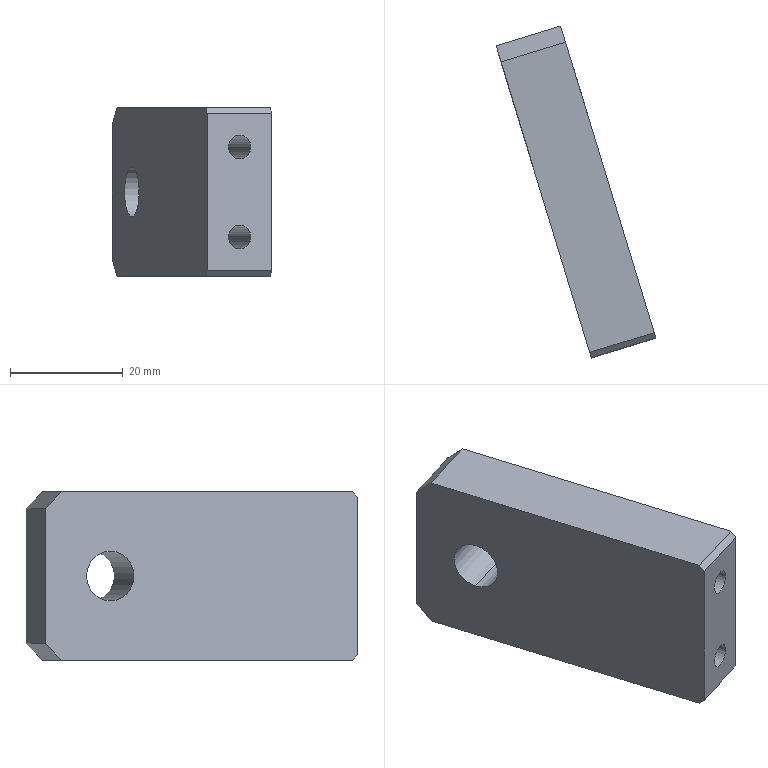Component | SolidWorks | V1ZHXTCylinderConnectionPlateSB1-1 | 1 solid | 20 faces | box 28.4 x 58.98 x 30 mm | volume 19536 mm3 | plane 10 | cylinder 6 | cone 4 | commonest cylinder face diameters 4.2 x4 8.8 x2
build123d program:
from build123d import *

# Parameters (mm, degrees)
SKETCH1_W               = 30
SKETCH1_H               = 12
BOSS_EXTRUDE1_DEPTH     = 58
M10X1_25_TAPPED_HOLE1_D = 8.8
CHAMFER1_SIZE           = 3
M5_TAPPED_HOLE1_D       = 4.2
M5_TAPPED_HOLE1_DEPTH   = 17.4
M5_TAPPED_HOLE1_TIP     = 1.262
CHAMFER2_SIZE           = 1


with BuildPart() as part:
    # Sketch1 → Boss-Extrude1 (new body)
    with BuildSketch(Plane(origin=(0, 0, 0), x_dir=(1, 0, 0), z_dir=(0, 1, 0))):
        Rectangle(SKETCH1_W, SKETCH1_H)
    extrude(amount=BOSS_EXTRUDE1_DEPTH)

    # M10x1.25 Tapped Hole1 (through all)
    with Locations(Plane.XY.offset(6)):
        with Locations((0, 46)):
            Hole(M10X1_25_TAPPED_HOLE1_D / 2)

    # Chamfer1
    chamfer1_edges = [part.edges().sort_by_distance(p)[0] for p in [
        (-15, 58, 0),
        (15, 58, 0),
    ]]
    chamfer(chamfer1_edges, length=CHAMFER1_SIZE)

    # M5 Tapped Hole1
    with Locations(Plane(origin=(0, 0, 0), x_dir=(-1, 0, 0), z_dir=(0, -1, 0))):
        with Locations((8, 0), (-8, 0)):
            Hole(M5_TAPPED_HOLE1_D / 2, depth=M5_TAPPED_HOLE1_DEPTH)
            with Locations((0, 0, -(M5_TAPPED_HOLE1_DEPTH + M5_TAPPED_HOLE1_TIP / 2))):  # 118° drill point
                Cone(0, M5_TAPPED_HOLE1_D / 2, M5_TAPPED_HOLE1_TIP, mode=Mode.SUBTRACT)

    # Chamfer2
    chamfer2_edges = [part.edges().sort_by_distance(p)[0] for p in [
        (-15, 0, 0),
        (15, 0, 0),
    ]]
    chamfer(chamfer2_edges, length=CHAMFER2_SIZE)


solid = part.part

# Placed as in the assembly
solid = solid.moved(Location((191.274, -170.356, 375.239), (90, -73.032, 90)))
STEP:
#1=COLOUR_RGB('',0.7922,0.8196,0.9333);
#2=FILL_AREA_STYLE_COLOUR('',#1);
#3=FILL_AREA_STYLE('',(#2));
#4=SURFACE_STYLE_FILL_AREA(#3);
#5=SURFACE_SIDE_STYLE('',(#4));
#6=SURFACE_STYLE_USAGE(.BOTH.,#5);
#7=PRESENTATION_STYLE_ASSIGNMENT((#6));
#8=CARTESIAN_POINT('',(7.41,-6.028,15.088));
#9=VERTEX_POINT('',#8);
#10=CARTESIAN_POINT('',(7.251,-6.076,15.088));
#11=VERTEX_POINT('',#10);
#12=CARTESIAN_POINT('',(7.331,-6.052,15.088));
#13=DIRECTION('',(0.2918,-0.9565,-0.));
#14=DIRECTION('',(-0.9565,-0.2918,-0.));
#15=AXIS2_PLACEMENT_3D('',#12,#13,#14);
#16=CIRCLE('',#15,0.08268);
#17=EDGE_CURVE('',#9,#11,#16,.T.);
#18=ORIENTED_EDGE('',*,*,#17,.F.);
#19=CARTESIAN_POINT('',(7.61,-6.683,15.088));
#20=VERTEX_POINT('',#19);
#21=CARTESIAN_POINT('',(7.61,-6.683,15.088));
#22=DIRECTION('',(0.2918,-0.9565,-0.));
#23=VECTOR('',#22,39.37);
#24=LINE('',#21,#23);
#25=EDGE_CURVE('',#9,#20,#24,.T.);
#26=ORIENTED_EDGE('',*,*,#25,.T.);
#27=CARTESIAN_POINT('',(7.451,-6.731,15.088));
#28=VERTEX_POINT('',#27);
#29=CARTESIAN_POINT('',(7.53,-6.707,15.088));
#30=DIRECTION('',(0.2918,-0.9565,-0.));
#31=DIRECTION('',(-0.9565,-0.2918,-0.));
#32=AXIS2_PLACEMENT_3D('',#29,#30,#31);
#33=CIRCLE('',#32,0.08268);
#34=EDGE_CURVE('',#20,#28,#33,.T.);
#35=ORIENTED_EDGE('',*,*,#34,.T.);
#36=CARTESIAN_POINT('',(7.451,-6.731,15.088));
#37=DIRECTION('',(0.2918,-0.9565,-0.));
#38=VECTOR('',#37,39.37);
#39=LINE('',#36,#38);
#40=EDGE_CURVE('',#11,#28,#39,.T.);
#41=ORIENTED_EDGE('',*,*,#40,.F.);
#42=EDGE_LOOP('',(#18,#26,#35,#41));
#43=FACE_OUTER_BOUND('',#42,.T.);
#44=CARTESIAN_POINT('',(7.53,-6.707,15.088));
#45=DIRECTION('',(0.2918,-0.9565,-0.));
#46=DIRECTION('',(-0.9565,-0.2918,-0.));
#47=AXIS2_PLACEMENT_3D('',#44,#45,#46);
#48=CYLINDRICAL_SURFACE('',#47,0.08268);
#49=ADVANCED_FACE('',(#43),#48,.F.);
#50=CARTESIAN_POINT('',(7.316,-6.004,15.088));
#51=VERTEX_POINT('',#50);
#52=CARTESIAN_POINT('',(7.251,-6.076,15.088));
#53=DIRECTION('',(-0.6696,-0.7428,-0.));
#54=VECTOR('',#53,39.37);
#55=LINE('',#52,#54);
#56=EDGE_CURVE('',#51,#11,#55,.T.);
#57=ORIENTED_EDGE('',*,*,#56,.F.);
#58=CARTESIAN_POINT('',(7.41,-6.028,15.088));
#59=DIRECTION('',(0.9702,-0.2425,-0.));
#60=VECTOR('',#59,39.37);
#61=LINE('',#58,#60);
#62=EDGE_CURVE('',#51,#9,#61,.T.);
#63=ORIENTED_EDGE('',*,*,#62,.T.);
#64=ORIENTED_EDGE('',*,*,#17,.T.);
#65=EDGE_LOOP('',(#57,#63,#64));
#66=FACE_OUTER_BOUND('',#65,.T.);
#67=CARTESIAN_POINT('',(7.331,-6.052,15.088));
#68=DIRECTION('',(0.2918,-0.9565,-0.));
#69=DIRECTION('',(-0.9565,-0.2918,-0.));
#70=AXIS2_PLACEMENT_3D('',#67,#68,#69);
#71=CONICAL_SURFACE('',#70,0.08268,1.03);
#72=ADVANCED_FACE('',(#66),#71,.F.);
#73=CARTESIAN_POINT('',(7.41,-6.028,14.458));
#74=VERTEX_POINT('',#73);
#75=CARTESIAN_POINT('',(7.251,-6.076,14.458));
#76=VERTEX_POINT('',#75);
#77=CARTESIAN_POINT('',(7.331,-6.052,14.458));
#78=DIRECTION('',(0.2918,-0.9565,-0.));
#79=DIRECTION('',(-0.9565,-0.2918,-0.));
#80=AXIS2_PLACEMENT_3D('',#77,#78,#79);
#81=CIRCLE('',#80,0.08268);
#82=EDGE_CURVE('',#74,#76,#81,.T.);
#83=ORIENTED_EDGE('',*,*,#82,.F.);
#84=CARTESIAN_POINT('',(7.61,-6.683,14.458));
#85=VERTEX_POINT('',#84);
#86=CARTESIAN_POINT('',(7.61,-6.683,14.458));
#87=DIRECTION('',(0.2918,-0.9565,-0.));
#88=VECTOR('',#87,39.37);
#89=LINE('',#86,#88);
#90=EDGE_CURVE('',#74,#85,#89,.T.);
#91=ORIENTED_EDGE('',*,*,#90,.T.);
#92=CARTESIAN_POINT('',(7.451,-6.731,14.458));
#93=VERTEX_POINT('',#92);
#94=CARTESIAN_POINT('',(7.53,-6.707,14.458));
#95=DIRECTION('',(0.2918,-0.9565,-0.));
#96=DIRECTION('',(-0.9565,-0.2918,-0.));
#97=AXIS2_PLACEMENT_3D('',#94,#95,#96);
#98=CIRCLE('',#97,0.08268);
#99=EDGE_CURVE('',#85,#93,#98,.T.);
#100=ORIENTED_EDGE('',*,*,#99,.T.);
#101=CARTESIAN_POINT('',(7.451,-6.731,14.458));
#102=DIRECTION('',(0.2918,-0.9565,-0.));
#103=VECTOR('',#102,39.37);
#104=LINE('',#101,#103);
#105=EDGE_CURVE('',#76,#93,#104,.T.);
#106=ORIENTED_EDGE('',*,*,#105,.F.);
#107=EDGE_LOOP('',(#83,#91,#100,#106));
#108=FACE_OUTER_BOUND('',#107,.T.);
#109=CARTESIAN_POINT('',(7.53,-6.707,14.458));
#110=DIRECTION('',(0.2918,-0.9565,-0.));
#111=DIRECTION('',(-0.9565,-0.2918,-0.));
#112=AXIS2_PLACEMENT_3D('',#109,#110,#111);
#113=CYLINDRICAL_SURFACE('',#112,0.08268);
#114=ADVANCED_FACE('',(#108),#113,.F.);
#115=CARTESIAN_POINT('',(7.316,-6.004,14.458));
#116=VERTEX_POINT('',#115);
#117=CARTESIAN_POINT('',(7.251,-6.076,14.458));
#118=DIRECTION('',(-0.6696,-0.7428,-0.));
#119=VECTOR('',#118,39.37);
#120=LINE('',#117,#119);
#121=EDGE_CURVE('',#116,#76,#120,.T.);
#122=ORIENTED_EDGE('',*,*,#121,.F.);
#123=CARTESIAN_POINT('',(7.41,-6.028,14.458));
#124=DIRECTION('',(0.9702,-0.2425,-0.));
#125=VECTOR('',#124,39.37);
#126=LINE('',#123,#125);
#127=EDGE_CURVE('',#116,#74,#126,.T.);
#128=ORIENTED_EDGE('',*,*,#127,.T.);
#129=ORIENTED_EDGE('',*,*,#82,.T.);
#130=EDGE_LOOP('',(#122,#128,#129));
#131=FACE_OUTER_BOUND('',#130,.T.);
#132=CARTESIAN_POINT('',(7.331,-6.052,14.458));
#133=DIRECTION('',(0.2918,-0.9565,-0.));
#134=DIRECTION('',(-0.9565,-0.2918,-0.));
#135=AXIS2_PLACEMENT_3D('',#132,#133,#134);
#136=CONICAL_SURFACE('',#135,0.08268,1.03);
#137=ADVANCED_FACE('',(#131),#136,.F.);
#138=CARTESIAN_POINT('',(6.776,-5.044,14.946));
#139=VERTEX_POINT('',#138);
#140=CARTESIAN_POINT('',(6.776,-5.044,14.6));
#141=VERTEX_POINT('',#140);
#142=CARTESIAN_POINT('',(6.776,-5.044,14.773));
#143=DIRECTION('',(0.9565,0.2918,0.));
#144=DIRECTION('',(0.,0.,-1.));
#145=AXIS2_PLACEMENT_3D('',#142,#143,#144);
#146=CIRCLE('',#145,0.1732);
#147=EDGE_CURVE('',#139,#141,#146,.T.);
#148=ORIENTED_EDGE('',*,*,#147,.F.);
#149=CARTESIAN_POINT('',(7.228,-4.906,14.946));
#150=VERTEX_POINT('',#149);
#151=CARTESIAN_POINT('',(7.228,-4.906,14.946));
#152=DIRECTION('',(0.9565,0.2918,0.));
#153=VECTOR('',#152,39.37);
#154=LINE('',#151,#153);
#155=EDGE_CURVE('',#139,#150,#154,.T.);
#156=ORIENTED_EDGE('',*,*,#155,.T.);
#157=CARTESIAN_POINT('',(7.228,-4.906,14.6));
#158=VERTEX_POINT('',#157);
#159=CARTESIAN_POINT('',(7.228,-4.906,14.773));
#160=DIRECTION('',(0.9565,0.2918,0.));
#161=DIRECTION('',(0.,0.,-1.));
#162=AXIS2_PLACEMENT_3D('',#159,#160,#161);
#163=CIRCLE('',#162,0.1732);
#164=EDGE_CURVE('',#150,#158,#163,.T.);
#165=ORIENTED_EDGE('',*,*,#164,.T.);
#166=CARTESIAN_POINT('',(7.228,-4.906,14.6));
#167=DIRECTION('',(0.9565,0.2918,0.));
#168=VECTOR('',#167,39.37);
#169=LINE('',#166,#168);
#170=EDGE_CURVE('',#141,#158,#169,.T.);
#171=ORIENTED_EDGE('',*,*,#170,.F.);
#172=EDGE_LOOP('',(#148,#156,#165,#171));
#173=FACE_OUTER_BOUND('',#172,.T.);
#174=CARTESIAN_POINT('',(7.228,-4.906,14.773));
#175=DIRECTION('',(0.9565,0.2918,0.));
#176=DIRECTION('',(0.,0.,-1.));
#177=AXIS2_PLACEMENT_3D('',#174,#175,#176);
#178=CYLINDRICAL_SURFACE('',#177,0.1732);
#179=ADVANCED_FACE('',(#173),#178,.F.);
#180=CARTESIAN_POINT('',(7.124,-4.567,14.183));
#181=VERTEX_POINT('',#180);
#182=CARTESIAN_POINT('',(7.745,-6.6,14.183));
#183=VERTEX_POINT('',#182);
#184=CARTESIAN_POINT('',(7.09,-4.454,14.183));
#185=DIRECTION('',(0.2918,-0.9565,-0.));
#186=VECTOR('',#185,39.37);
#187=LINE('',#184,#186);
#188=EDGE_CURVE('',#181,#183,#187,.T.);
#189=ORIENTED_EDGE('',*,*,#188,.T.);
#190=CARTESIAN_POINT('',(7.293,-6.738,14.183));
#191=VERTEX_POINT('',#190);
#192=CARTESIAN_POINT('',(7.293,-6.738,14.183));
#193=DIRECTION('',(-0.9565,-0.2918,-0.));
#194=VECTOR('',#193,39.37);
#195=LINE('',#192,#194);
#196=EDGE_CURVE('',#183,#191,#195,.T.);
#197=ORIENTED_EDGE('',*,*,#196,.T.);
#198=CARTESIAN_POINT('',(6.673,-4.705,14.183));
#199=VERTEX_POINT('',#198);
#200=CARTESIAN_POINT('',(6.638,-4.592,14.183));
#201=DIRECTION('',(0.2918,-0.9565,-0.));
#202=VECTOR('',#201,39.37);
#203=LINE('',#200,#202);
#204=EDGE_CURVE('',#199,#191,#203,.T.);
#205=ORIENTED_EDGE('',*,*,#204,.F.);
#206=CARTESIAN_POINT('',(7.124,-4.567,14.183));
#207=DIRECTION('',(0.9565,0.2918,0.));
#208=VECTOR('',#207,39.37);
#209=LINE('',#206,#208);
#210=EDGE_CURVE('',#199,#181,#209,.T.);
#211=ORIENTED_EDGE('',*,*,#210,.T.);
#212=EDGE_LOOP('',(#189,#197,#205,#211));
#213=FACE_OUTER_BOUND('',#212,.T.);
#214=CARTESIAN_POINT('',(7.09,-4.454,14.183));
#215=DIRECTION('',(-0.,-0.,1.));
#216=DIRECTION('',(0.9565,0.2918,0.));
#217=AXIS2_PLACEMENT_3D('',#214,#215,#216);
#218=PLANE('',#217);
#219=ADVANCED_FACE('',(#213),#218,.F.);
#220=CARTESIAN_POINT('',(6.776,-5.044,14.773));
#221=DIRECTION('',(0.9565,0.2918,0.));
#222=DIRECTION('',(0.,0.,-1.));
#223=AXIS2_PLACEMENT_3D('',#220,#221,#222);
#224=CIRCLE('',#223,0.1732);
#225=EDGE_CURVE('',#141,#139,#224,.T.);
#226=ORIENTED_EDGE('',*,*,#225,.T.);
#227=ORIENTED_EDGE('',*,*,#147,.T.);
#228=EDGE_LOOP('',(#226,#227));
#229=FACE_BOUND('',#228,.T.);
#230=CARTESIAN_POINT('',(7.305,-6.776,14.222));
#231=VERTEX_POINT('',#230);
#232=CARTESIAN_POINT('',(7.305,-6.776,15.324));
#233=VERTEX_POINT('',#232);
#234=CARTESIAN_POINT('',(7.305,-6.776,15.364));
#235=DIRECTION('',(-0.,-0.,1.));
#236=VECTOR('',#235,39.37);
#237=LINE('',#234,#236);
#238=EDGE_CURVE('',#231,#233,#237,.T.);
#239=ORIENTED_EDGE('',*,*,#238,.T.);
#240=CARTESIAN_POINT('',(7.293,-6.738,15.364));
#241=VERTEX_POINT('',#240);
#242=CARTESIAN_POINT('',(7.293,-6.738,15.364));
#243=DIRECTION('',(-0.2064,0.6763,0.7071));
#244=VECTOR('',#243,39.37);
#245=LINE('',#242,#244);
#246=EDGE_CURVE('',#233,#241,#245,.T.);
#247=ORIENTED_EDGE('',*,*,#246,.T.);
#248=CARTESIAN_POINT('',(6.673,-4.705,15.364));
#249=VERTEX_POINT('',#248);
#250=CARTESIAN_POINT('',(6.638,-4.592,15.364));
#251=DIRECTION('',(0.2918,-0.9565,-0.));
#252=VECTOR('',#251,39.37);
#253=LINE('',#250,#252);
#254=EDGE_CURVE('',#249,#241,#253,.T.);
#255=ORIENTED_EDGE('',*,*,#254,.F.);
#256=CARTESIAN_POINT('',(6.638,-4.592,15.246));
#257=VERTEX_POINT('',#256);
#258=CARTESIAN_POINT('',(6.638,-4.592,15.246));
#259=DIRECTION('',(-0.2064,0.6763,-0.7071));
#260=VECTOR('',#259,39.37);
#261=LINE('',#258,#260);
#262=EDGE_CURVE('',#249,#257,#261,.T.);
#263=ORIENTED_EDGE('',*,*,#262,.T.);
#264=CARTESIAN_POINT('',(6.638,-4.592,14.301));
#265=VERTEX_POINT('',#264);
#266=CARTESIAN_POINT('',(6.638,-4.592,15.364));
#267=DIRECTION('',(-0.,-0.,1.));
#268=VECTOR('',#267,39.37);
#269=LINE('',#266,#268);
#270=EDGE_CURVE('',#265,#257,#269,.T.);
#271=ORIENTED_EDGE('',*,*,#270,.F.);
#272=CARTESIAN_POINT('',(6.638,-4.592,14.301));
#273=DIRECTION('',(0.2064,-0.6763,-0.7071));
#274=VECTOR('',#273,39.37);
#275=LINE('',#272,#274);
#276=EDGE_CURVE('',#265,#199,#275,.T.);
#277=ORIENTED_EDGE('',*,*,#276,.T.);
#278=ORIENTED_EDGE('',*,*,#204,.T.);
#279=CARTESIAN_POINT('',(7.293,-6.738,14.183));
#280=DIRECTION('',(0.2064,-0.6763,0.7071));
#281=VECTOR('',#280,39.37);
#282=LINE('',#279,#281);
#283=EDGE_CURVE('',#191,#231,#282,.T.);
#284=ORIENTED_EDGE('',*,*,#283,.T.);
#285=EDGE_LOOP('',(#239,#247,#255,#263,#271,#277,#278,#284));
#286=FACE_OUTER_BOUND('',#285,.T.);
#287=CARTESIAN_POINT('',(6.638,-4.592,15.364));
#288=DIRECTION('',(0.9565,0.2918,0.));
#289=DIRECTION('',(0.,0.,-1.));
#290=AXIS2_PLACEMENT_3D('',#287,#288,#289);
#291=PLANE('',#290);
#292=ADVANCED_FACE('',(#229,#286),#291,.F.);
#293=ORIENTED_EDGE('',*,*,#254,.T.);
#294=CARTESIAN_POINT('',(7.745,-6.6,15.364));
#295=VERTEX_POINT('',#294);
#296=CARTESIAN_POINT('',(7.745,-6.6,15.364));
#297=DIRECTION('',(0.9565,0.2918,0.));
#298=VECTOR('',#297,39.37);
#299=LINE('',#296,#298);
#300=EDGE_CURVE('',#241,#295,#299,.T.);
#301=ORIENTED_EDGE('',*,*,#300,.T.);
#302=CARTESIAN_POINT('',(7.124,-4.567,15.364));
#303=VERTEX_POINT('',#302);
#304=CARTESIAN_POINT('',(7.09,-4.454,15.364));
#305=DIRECTION('',(0.2918,-0.9565,-0.));
#306=VECTOR('',#305,39.37);
#307=LINE('',#304,#306);
#308=EDGE_CURVE('',#303,#295,#307,.T.);
#309=ORIENTED_EDGE('',*,*,#308,.F.);
#310=CARTESIAN_POINT('',(7.124,-4.567,15.364));
#311=DIRECTION('',(-0.9565,-0.2918,-0.));
#312=VECTOR('',#311,39.37);
#313=LINE('',#310,#312);
#314=EDGE_CURVE('',#303,#249,#313,.T.);
#315=ORIENTED_EDGE('',*,*,#314,.T.);
#316=EDGE_LOOP('',(#293,#301,#309,#315));
#317=FACE_OUTER_BOUND('',#316,.T.);
#318=CARTESIAN_POINT('',(7.09,-4.454,15.364));
#319=DIRECTION('',(0.,0.,-1.));
#320=DIRECTION('',(-0.9565,-0.2918,-0.));
#321=AXIS2_PLACEMENT_3D('',#318,#319,#320);
#322=PLANE('',#321);
#323=ADVANCED_FACE('',(#317),#322,.F.);
#324=CARTESIAN_POINT('',(7.228,-4.906,14.773));
#325=DIRECTION('',(0.9565,0.2918,0.));
#326=DIRECTION('',(0.,0.,-1.));
#327=AXIS2_PLACEMENT_3D('',#324,#325,#326);
#328=CIRCLE('',#327,0.1732);
#329=EDGE_CURVE('',#158,#150,#328,.T.);
#330=ORIENTED_EDGE('',*,*,#329,.F.);
#331=ORIENTED_EDGE('',*,*,#164,.F.);
#332=EDGE_LOOP('',(#330,#331));
#333=FACE_BOUND('',#332,.T.);
#334=ORIENTED_EDGE('',*,*,#308,.T.);
#335=CARTESIAN_POINT('',(7.756,-6.638,15.324));
#336=VERTEX_POINT('',#335);
#337=CARTESIAN_POINT('',(7.745,-6.6,15.364));
#338=DIRECTION('',(0.2064,-0.6763,-0.7071));
#339=VECTOR('',#338,39.37);
#340=LINE('',#337,#339);
#341=EDGE_CURVE('',#295,#336,#340,.T.);
#342=ORIENTED_EDGE('',*,*,#341,.T.);
#343=CARTESIAN_POINT('',(7.756,-6.638,14.222));
#344=VERTEX_POINT('',#343);
#345=CARTESIAN_POINT('',(7.756,-6.638,15.364));
#346=DIRECTION('',(0.,0.,-1.));
#347=VECTOR('',#346,39.37);
#348=LINE('',#345,#347);
#349=EDGE_CURVE('',#336,#344,#348,.T.);
#350=ORIENTED_EDGE('',*,*,#349,.T.);
#351=CARTESIAN_POINT('',(7.745,-6.6,14.183));
#352=DIRECTION('',(-0.2064,0.6763,-0.7071));
#353=VECTOR('',#352,39.37);
#354=LINE('',#351,#353);
#355=EDGE_CURVE('',#344,#183,#354,.T.);
#356=ORIENTED_EDGE('',*,*,#355,.T.);
#357=ORIENTED_EDGE('',*,*,#188,.F.);
#358=CARTESIAN_POINT('',(7.09,-4.454,14.301));
#359=VERTEX_POINT('',#358);
#360=CARTESIAN_POINT('',(7.09,-4.454,14.301));
#361=DIRECTION('',(-0.2064,0.6763,0.7071));
#362=VECTOR('',#361,39.37);
#363=LINE('',#360,#362);
#364=EDGE_CURVE('',#181,#359,#363,.T.);
#365=ORIENTED_EDGE('',*,*,#364,.T.);
#366=CARTESIAN_POINT('',(7.09,-4.454,15.246));
#367=VERTEX_POINT('',#366);
#368=CARTESIAN_POINT('',(7.09,-4.454,15.364));
#369=DIRECTION('',(0.,0.,-1.));
#370=VECTOR('',#369,39.37);
#371=LINE('',#368,#370);
#372=EDGE_CURVE('',#367,#359,#371,.T.);
#373=ORIENTED_EDGE('',*,*,#372,.F.);
#374=CARTESIAN_POINT('',(7.09,-4.454,15.246));
#375=DIRECTION('',(0.2064,-0.6763,0.7071));
#376=VECTOR('',#375,39.37);
#377=LINE('',#374,#376);
#378=EDGE_CURVE('',#367,#303,#377,.T.);
#379=ORIENTED_EDGE('',*,*,#378,.T.);
#380=EDGE_LOOP('',(#334,#342,#350,#356,#357,#365,#373,#379));
#381=FACE_OUTER_BOUND('',#380,.T.);
#382=CARTESIAN_POINT('',(7.09,-4.454,15.364));
#383=DIRECTION('',(-0.9565,-0.2918,-0.));
#384=DIRECTION('',(-0.,-0.,1.));
#385=AXIS2_PLACEMENT_3D('',#382,#383,#384);
#386=PLANE('',#385);
#387=ADVANCED_FACE('',(#333,#381),#386,.F.);
#388=ORIENTED_EDGE('',*,*,#270,.T.);
#389=CARTESIAN_POINT('',(6.864,-4.523,15.246));
#390=DIRECTION('',(0.9565,0.2918,0.));
#391=VECTOR('',#390,39.37);
#392=LINE('',#389,#391);
#393=EDGE_CURVE('',#257,#367,#392,.T.);
#394=ORIENTED_EDGE('',*,*,#393,.T.);
#395=ORIENTED_EDGE('',*,*,#372,.T.);
#396=CARTESIAN_POINT('',(6.864,-4.523,14.301));
#397=DIRECTION('',(-0.9565,-0.2918,-0.));
#398=VECTOR('',#397,39.37);
#399=LINE('',#396,#398);
#400=EDGE_CURVE('',#359,#265,#399,.T.);
#401=ORIENTED_EDGE('',*,*,#400,.T.);
#402=EDGE_LOOP('',(#388,#394,#395,#401));
#403=FACE_OUTER_BOUND('',#402,.T.);
#404=CARTESIAN_POINT('',(6.864,-4.523,14.773));
#405=DIRECTION('',(0.2918,-0.9565,-0.));
#406=DIRECTION('',(-0.9565,-0.2918,-0.));
#407=AXIS2_PLACEMENT_3D('',#404,#405,#406);
#408=PLANE('',#407);
#409=ADVANCED_FACE('',(#403),#408,.F.);
#410=CARTESIAN_POINT('',(7.53,-6.707,15.088));
#411=DIRECTION('',(0.2918,-0.9565,-0.));
#412=DIRECTION('',(-0.9565,-0.2918,-0.));
#413=AXIS2_PLACEMENT_3D('',#410,#411,#412);
#414=CIRCLE('',#413,0.08268);
#415=EDGE_CURVE('',#28,#20,#414,.T.);
#416=ORIENTED_EDGE('',*,*,#415,.F.);
#417=ORIENTED_EDGE('',*,*,#34,.F.);
#418=EDGE_LOOP('',(#416,#417));
#419=FACE_BOUND('',#418,.T.);
#420=CARTESIAN_POINT('',(7.53,-6.707,14.458));
#421=DIRECTION('',(0.2918,-0.9565,-0.));
#422=DIRECTION('',(-0.9565,-0.2918,-0.));
#423=AXIS2_PLACEMENT_3D('',#420,#421,#422);
#424=CIRCLE('',#423,0.08268);
#425=EDGE_CURVE('',#93,#85,#424,.T.);
#426=ORIENTED_EDGE('',*,*,#425,.F.);
#427=ORIENTED_EDGE('',*,*,#99,.F.);
#428=EDGE_LOOP('',(#426,#427));
#429=FACE_BOUND('',#428,.T.);
#430=ORIENTED_EDGE('',*,*,#349,.F.);
#431=CARTESIAN_POINT('',(7.305,-6.776,15.324));
#432=DIRECTION('',(-0.9565,-0.2918,-0.));
#433=VECTOR('',#432,39.37);
#434=LINE('',#431,#433);
#435=EDGE_CURVE('',#336,#233,#434,.T.);
#436=ORIENTED_EDGE('',*,*,#435,.T.);
#437=ORIENTED_EDGE('',*,*,#238,.F.);
#438=CARTESIAN_POINT('',(7.756,-6.638,14.222));
#439=DIRECTION('',(0.9565,0.2918,0.));
#440=VECTOR('',#439,39.37);
#441=LINE('',#438,#440);
#442=EDGE_CURVE('',#231,#344,#441,.T.);
#443=ORIENTED_EDGE('',*,*,#442,.T.);
#444=EDGE_LOOP('',(#430,#436,#437,#443));
#445=FACE_OUTER_BOUND('',#444,.T.);
#446=CARTESIAN_POINT('',(7.53,-6.707,14.773));
#447=DIRECTION('',(0.2918,-0.9565,-0.));
#448=DIRECTION('',(-0.9565,-0.2918,-0.));
#449=AXIS2_PLACEMENT_3D('',#446,#447,#448);
#450=PLANE('',#449);
#451=ADVANCED_FACE('',(#419,#429,#445),#450,.T.);
#452=ORIENTED_EDGE('',*,*,#155,.F.);
#453=ORIENTED_EDGE('',*,*,#225,.F.);
#454=ORIENTED_EDGE('',*,*,#170,.T.);
#455=ORIENTED_EDGE('',*,*,#329,.T.);
#456=EDGE_LOOP('',(#452,#453,#454,#455));
#457=FACE_OUTER_BOUND('',#456,.T.);
#458=CARTESIAN_POINT('',(7.228,-4.906,14.773));
#459=DIRECTION('',(0.9565,0.2918,0.));
#460=DIRECTION('',(0.,0.,-1.));
#461=AXIS2_PLACEMENT_3D('',#458,#459,#460);
#462=CYLINDRICAL_SURFACE('',#461,0.1732);
#463=ADVANCED_FACE('',(#457),#462,.F.);
#464=ORIENTED_EDGE('',*,*,#262,.F.);
#465=ORIENTED_EDGE('',*,*,#314,.F.);
#466=ORIENTED_EDGE('',*,*,#378,.F.);
#467=ORIENTED_EDGE('',*,*,#393,.F.);
#468=EDGE_LOOP('',(#464,#465,#466,#467));
#469=FACE_OUTER_BOUND('',#468,.T.);
#470=CARTESIAN_POINT('',(6.864,-4.523,15.246));
#471=DIRECTION('',(0.2064,-0.6763,-0.7071));
#472=DIRECTION('',(0.9565,0.2918,0.));
#473=AXIS2_PLACEMENT_3D('',#470,#471,#472);
#474=PLANE('',#473);
#475=ADVANCED_FACE('',(#469),#474,.F.);
#476=ORIENTED_EDGE('',*,*,#364,.F.);
#477=ORIENTED_EDGE('',*,*,#210,.F.);
#478=ORIENTED_EDGE('',*,*,#276,.F.);
#479=ORIENTED_EDGE('',*,*,#400,.F.);
#480=EDGE_LOOP('',(#476,#477,#478,#479));
#481=FACE_OUTER_BOUND('',#480,.T.);
#482=CARTESIAN_POINT('',(6.864,-4.523,14.301));
#483=DIRECTION('',(0.2064,-0.6763,0.7071));
#484=DIRECTION('',(-0.9565,-0.2918,-0.));
#485=AXIS2_PLACEMENT_3D('',#482,#483,#484);
#486=PLANE('',#485);
#487=ADVANCED_FACE('',(#481),#486,.F.);
#488=ORIENTED_EDGE('',*,*,#127,.F.);
#489=ORIENTED_EDGE('',*,*,#121,.T.);
#490=CARTESIAN_POINT('',(7.331,-6.052,14.458));
#491=DIRECTION('',(0.2918,-0.9565,-0.));
#492=DIRECTION('',(-0.9565,-0.2918,-0.));
#493=AXIS2_PLACEMENT_3D('',#490,#491,#492);
#494=CIRCLE('',#493,0.08268);
#495=EDGE_CURVE('',#76,#74,#494,.T.);
#496=ORIENTED_EDGE('',*,*,#495,.T.);
#497=EDGE_LOOP('',(#488,#489,#496));
#498=FACE_OUTER_BOUND('',#497,.T.);
#499=CARTESIAN_POINT('',(7.331,-6.052,14.458));
#500=DIRECTION('',(0.2918,-0.9565,-0.));
#501=DIRECTION('',(-0.9565,-0.2918,-0.));
#502=AXIS2_PLACEMENT_3D('',#499,#500,#501);
#503=CONICAL_SURFACE('',#502,0.08268,1.03);
#504=ADVANCED_FACE('',(#498),#503,.F.);
#505=ORIENTED_EDGE('',*,*,#90,.F.);
#506=ORIENTED_EDGE('',*,*,#495,.F.);
#507=ORIENTED_EDGE('',*,*,#105,.T.);
#508=ORIENTED_EDGE('',*,*,#425,.T.);
#509=EDGE_LOOP('',(#505,#506,#507,#508));
#510=FACE_OUTER_BOUND('',#509,.T.);
#511=CARTESIAN_POINT('',(7.53,-6.707,14.458));
#512=DIRECTION('',(0.2918,-0.9565,-0.));
#513=DIRECTION('',(-0.9565,-0.2918,-0.));
#514=AXIS2_PLACEMENT_3D('',#511,#512,#513);
#515=CYLINDRICAL_SURFACE('',#514,0.08268);
#516=ADVANCED_FACE('',(#510),#515,.F.);
#517=ORIENTED_EDGE('',*,*,#62,.F.);
#518=ORIENTED_EDGE('',*,*,#56,.T.);
#519=CARTESIAN_POINT('',(7.331,-6.052,15.088));
#520=DIRECTION('',(0.2918,-0.9565,-0.));
#521=DIRECTION('',(-0.9565,-0.2918,-0.));
#522=AXIS2_PLACEMENT_3D('',#519,#520,#521);
#523=CIRCLE('',#522,0.08268);
#524=EDGE_CURVE('',#11,#9,#523,.T.);
#525=ORIENTED_EDGE('',*,*,#524,.T.);
#526=EDGE_LOOP('',(#517,#518,#525));
#527=FACE_OUTER_BOUND('',#526,.T.);
#528=CARTESIAN_POINT('',(7.331,-6.052,15.088));
#529=DIRECTION('',(0.2918,-0.9565,-0.));
#530=DIRECTION('',(-0.9565,-0.2918,-0.));
#531=AXIS2_PLACEMENT_3D('',#528,#529,#530);
#532=CONICAL_SURFACE('',#531,0.08268,1.03);
#533=ADVANCED_FACE('',(#527),#532,.F.);
#534=ORIENTED_EDGE('',*,*,#25,.F.);
#535=ORIENTED_EDGE('',*,*,#524,.F.);
#536=ORIENTED_EDGE('',*,*,#40,.T.);
#537=ORIENTED_EDGE('',*,*,#415,.T.);
#538=EDGE_LOOP('',(#534,#535,#536,#537));
#539=FACE_OUTER_BOUND('',#538,.T.);
#540=CARTESIAN_POINT('',(7.53,-6.707,15.088));
#541=DIRECTION('',(0.2918,-0.9565,-0.));
#542=DIRECTION('',(-0.9565,-0.2918,-0.));
#543=AXIS2_PLACEMENT_3D('',#540,#541,#542);
#544=CYLINDRICAL_SURFACE('',#543,0.08268);
#545=ADVANCED_FACE('',(#539),#544,.F.);
#546=ORIENTED_EDGE('',*,*,#246,.F.);
#547=ORIENTED_EDGE('',*,*,#435,.F.);
#548=ORIENTED_EDGE('',*,*,#341,.F.);
#549=ORIENTED_EDGE('',*,*,#300,.F.);
#550=EDGE_LOOP('',(#546,#547,#548,#549));
#551=FACE_OUTER_BOUND('',#550,.T.);
#552=CARTESIAN_POINT('',(7.745,-6.6,15.364));
#553=DIRECTION('',(0.2064,-0.6763,0.7071));
#554=DIRECTION('',(-0.9565,-0.2918,-0.));
#555=AXIS2_PLACEMENT_3D('',#552,#553,#554);
#556=PLANE('',#555);
#557=ADVANCED_FACE('',(#551),#556,.T.);
#558=ORIENTED_EDGE('',*,*,#355,.F.);
#559=ORIENTED_EDGE('',*,*,#442,.F.);
#560=ORIENTED_EDGE('',*,*,#283,.F.);
#561=ORIENTED_EDGE('',*,*,#196,.F.);
#562=EDGE_LOOP('',(#558,#559,#560,#561));
#563=FACE_OUTER_BOUND('',#562,.T.);
#564=CARTESIAN_POINT('',(7.745,-6.6,14.183));
#565=DIRECTION('',(0.2064,-0.6763,-0.7071));
#566=DIRECTION('',(0.9565,0.2918,0.));
#567=AXIS2_PLACEMENT_3D('',#564,#565,#566);
#568=PLANE('',#567);
#569=ADVANCED_FACE('',(#563),#568,.T.);
#570=CLOSED_SHELL('',(#49,#72,#114,#137,#179,#219,#292,#323,#387,#409,#451,#463,#475,#487,#504,#516,#533,#545,#557,#569));
#571=MANIFOLD_SOLID_BREP('',#570);
#572=STYLED_ITEM('',(#7),#571);
#573=PRESENTATION_LAYER_ASSIGNMENT('','',(#572));
#574=CARTESIAN_POINT('',(0.,0.,0.));
#575=DIRECTION('',(0.,0.,1.));
#576=DIRECTION('',(1.,0.,0.));
#577=AXIS2_PLACEMENT_3D('',#574,#575,#576);
#578=(LENGTH_UNIT()NAMED_UNIT(*)SI_UNIT($,.METRE.));
#579=LENGTH_MEASURE_WITH_UNIT(LENGTH_MEASURE(0.0254),#578);
#580=DIMENSIONAL_EXPONENTS(1.,0.,0.,0.,0.,0.,0.);
#581=(CONVERSION_BASED_UNIT('',#579)LENGTH_UNIT()NAMED_UNIT(#580));
#582=UNCERTAINTY_MEASURE_WITH_UNIT(LENGTH_MEASURE(0.00001),#581,'','');
#583=(NAMED_UNIT(*)PLANE_ANGLE_UNIT()SI_UNIT($,.RADIAN.));
#584=(NAMED_UNIT(*)SI_UNIT($,.STERADIAN.)SOLID_ANGLE_UNIT());
#585=(GEOMETRIC_REPRESENTATION_CONTEXT(3)GLOBAL_UNCERTAINTY_ASSIGNED_CONTEXT((#582))GLOBAL_UNIT_ASSIGNED_CONTEXT((#581,#583,#584))REPRESENTATION_CONTEXT('',''));
#586=ADVANCED_BREP_SHAPE_REPRESENTATION('',(#571,#577),#585);
#587=(LENGTH_UNIT()NAMED_UNIT(*)SI_UNIT($,.METRE.));
#588=LENGTH_MEASURE_WITH_UNIT(LENGTH_MEASURE(0.0254),#587);
#589=DIMENSIONAL_EXPONENTS(1.,0.,0.,0.,0.,0.,0.);
#590=(CONVERSION_BASED_UNIT('',#588)LENGTH_UNIT()NAMED_UNIT(#589));
#591=UNCERTAINTY_MEASURE_WITH_UNIT(LENGTH_MEASURE(0.00001),#590,'','');
#592=(NAMED_UNIT(*)PLANE_ANGLE_UNIT()SI_UNIT($,.RADIAN.));
#593=(NAMED_UNIT(*)SI_UNIT($,.STERADIAN.)SOLID_ANGLE_UNIT());
#594=(GEOMETRIC_REPRESENTATION_CONTEXT(3)GLOBAL_UNCERTAINTY_ASSIGNED_CONTEXT((#591))GLOBAL_UNIT_ASSIGNED_CONTEXT((#590,#592,#593))REPRESENTATION_CONTEXT('',''));
#595=MECHANICAL_DESIGN_GEOMETRIC_PRESENTATION_REPRESENTATION('',(#572),#594);